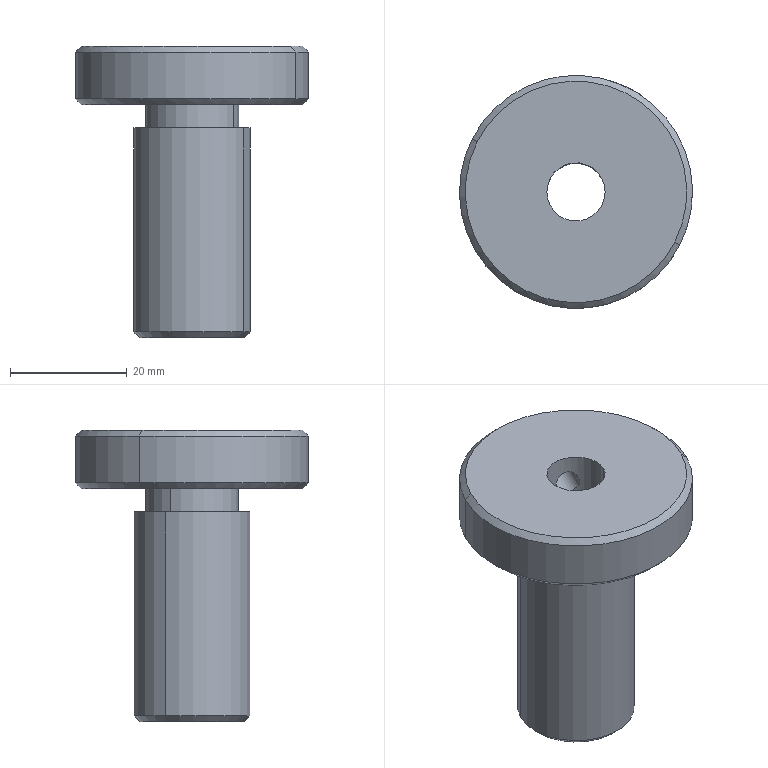Component | SolidWorks | AdjustingScrew-1 | 1 solid | 20 faces | box 40 x 40 x 50 mm | volume 20390 mm3 | cylinder 10 | cone 6 | plane 4 | commonest cylinder face diameters 4.2 x2 10 x2 40 x2 16 x2 20 x2
build123d program:
from build123d import *

# Parameters (mm, degrees)
F_10_0_10_DIAMETER_HOLE1_D = 10
SKETCH4_W                  = 2.1
SKETCH4_H                  = 15.462


with BuildPart() as part:
    # Sketch1 → Revolve1 (revolve)
    with BuildSketch(Plane.XY, mode=Mode.PRIVATE) as revolve1_sk:
        Polygon((-50, 9), (-50, 0), (0, 0), (0, 19), (-1, 20), (-9, 20), (-10, 19), (-10, 8), (-14, 8), (-14, 10), (-49, 10), align=None)
    revolve(revolve1_sk.sketch.rotate(Axis((-50, 0, 0), (1, 0, 0)), 270), axis=Axis((-50, 0, 0), (1, 0, 0)))

    # 10.0 _10_ Diameter Hole1 (through all)
    with Locations(Plane.ZY.offset(50)):
        with Locations((0, 0)):
            Hole(F_10_0_10_DIAMETER_HOLE1_D / 2)

    # Sketch4 → 4.2 _4.2_ Diameter Hole1 (revolve, cut)
    with BuildSketch(Plane(origin=(-5, 4.538, 0), x_dir=(0, 0, -1), z_dir=(1, 0, 0))):
        with Locations((1.05, 7.731)):
            Rectangle(SKETCH4_W, SKETCH4_H)
    revolve(axis=Axis((-5, -1.812, 0), (0, 1, 0)), mode=Mode.SUBTRACT)


solid = part.part

# Placed as in the assembly
solid = solid.moved(Location((376.258, 489.105, 284.94), (-90, -63.116, -90)))
STEP:
#1=COLOUR_RGB('',0.7922,0.8196,0.9333);
#2=FILL_AREA_STYLE_COLOUR('',#1);
#3=FILL_AREA_STYLE('',(#2));
#4=SURFACE_STYLE_FILL_AREA(#3);
#5=SURFACE_SIDE_STYLE('',(#4));
#6=SURFACE_STYLE_USAGE(.BOTH.,#5);
#7=PRESENTATION_STYLE_ASSIGNMENT((#6));
#8=CARTESIAN_POINT('',(15.241,19.917,11.021));
#9=VERTEX_POINT('',#8);
#10=CARTESIAN_POINT('',(15.094,19.992,11.021));
#11=VERTEX_POINT('',#10);
#12=CARTESIAN_POINT('',(15.241,19.917,11.021));
#13=CARTESIAN_POINT('',(15.241,19.917,11.016));
#14=CARTESIAN_POINT('',(15.241,19.917,11.01));
#15=CARTESIAN_POINT('',(15.239,19.919,11.));
#16=CARTESIAN_POINT('',(15.238,19.919,10.995));
#17=CARTESIAN_POINT('',(15.234,19.922,10.985));
#18=CARTESIAN_POINT('',(15.232,19.923,10.98));
#19=CARTESIAN_POINT('',(15.227,19.926,10.971));
#20=CARTESIAN_POINT('',(15.224,19.928,10.967));
#21=CARTESIAN_POINT('',(15.217,19.932,10.959));
#22=CARTESIAN_POINT('',(15.214,19.934,10.956));
#23=CARTESIAN_POINT('',(15.206,19.939,10.95));
#24=CARTESIAN_POINT('',(15.202,19.941,10.947));
#25=CARTESIAN_POINT('',(15.193,19.946,10.943));
#26=CARTESIAN_POINT('',(15.188,19.948,10.941));
#27=CARTESIAN_POINT('',(15.179,19.953,10.939));
#28=CARTESIAN_POINT('',(15.174,19.956,10.939));
#29=CARTESIAN_POINT('',(15.16,19.963,10.939));
#30=CARTESIAN_POINT('',(15.15,19.968,10.941));
#31=CARTESIAN_POINT('',(15.132,19.976,10.949));
#32=CARTESIAN_POINT('',(15.123,19.98,10.955));
#33=CARTESIAN_POINT('',(15.113,19.984,10.967));
#34=CARTESIAN_POINT('',(15.109,19.986,10.971));
#35=CARTESIAN_POINT('',(15.104,19.988,10.98));
#36=CARTESIAN_POINT('',(15.102,19.989,10.985));
#37=CARTESIAN_POINT('',(15.098,19.99,10.995));
#38=CARTESIAN_POINT('',(15.096,19.991,11.));
#39=CARTESIAN_POINT('',(15.094,19.992,11.01));
#40=CARTESIAN_POINT('',(15.094,19.992,11.016));
#41=CARTESIAN_POINT('',(15.094,19.992,11.021));
#42=B_SPLINE_CURVE_WITH_KNOTS('',3,(#12,#13,#14,#15,#16,#17,#18,#19,#20,#21,#22,#23,#24,#25,#26,#27,#28,#29,#30,#31,#32,#33,#34,#35,#36,#37,#38,#39,#40,#41),.UNSPECIFIED.,.F.,.F.,(4,2,2,2,2,2,2,2,2,2,2,2,2,2,4),(0.003286,0.003696,0.004107,0.004518,0.004928,0.005339,0.00575,0.00616,0.006571,0.007392,0.008213,0.008624,0.009035,0.009445,0.009856),.UNSPECIFIED.);
#43=EDGE_CURVE('',#9,#11,#42,.T.);
#44=ORIENTED_EDGE('',*,*,#43,.T.);
#45=CARTESIAN_POINT('',(14.82,19.453,11.021));
#46=VERTEX_POINT('',#45);
#47=CARTESIAN_POINT('',(14.82,19.453,11.021));
#48=DIRECTION('',(-0.4522,-0.8919,-0.));
#49=VECTOR('',#48,39.37);
#50=LINE('',#47,#49);
#51=EDGE_CURVE('',#11,#46,#50,.T.);
#52=ORIENTED_EDGE('',*,*,#51,.T.);
#53=CARTESIAN_POINT('',(14.968,19.378,11.021));
#54=VERTEX_POINT('',#53);
#55=CARTESIAN_POINT('',(14.968,19.378,11.021));
#56=CARTESIAN_POINT('',(14.968,19.378,11.016));
#57=CARTESIAN_POINT('',(14.967,19.379,11.01));
#58=CARTESIAN_POINT('',(14.966,19.38,11.));
#59=CARTESIAN_POINT('',(14.965,19.382,10.994));
#60=CARTESIAN_POINT('',(14.962,19.385,10.984));
#61=CARTESIAN_POINT('',(14.96,19.387,10.98));
#62=CARTESIAN_POINT('',(14.956,19.392,10.971));
#63=CARTESIAN_POINT('',(14.953,19.395,10.967));
#64=CARTESIAN_POINT('',(14.945,19.403,10.955));
#65=CARTESIAN_POINT('',(14.938,19.409,10.949));
#66=CARTESIAN_POINT('',(14.926,19.418,10.943));
#67=CARTESIAN_POINT('',(14.921,19.421,10.941));
#68=CARTESIAN_POINT('',(14.912,19.427,10.939));
#69=CARTESIAN_POINT('',(14.907,19.429,10.939));
#70=CARTESIAN_POINT('',(14.897,19.434,10.939));
#71=CARTESIAN_POINT('',(14.892,19.436,10.939));
#72=CARTESIAN_POINT('',(14.883,19.44,10.941));
#73=CARTESIAN_POINT('',(14.878,19.442,10.943));
#74=CARTESIAN_POINT('',(14.868,19.445,10.947));
#75=CARTESIAN_POINT('',(14.863,19.447,10.95));
#76=CARTESIAN_POINT('',(14.854,19.449,10.956));
#77=CARTESIAN_POINT('',(14.85,19.45,10.959));
#78=CARTESIAN_POINT('',(14.842,19.451,10.967));
#79=CARTESIAN_POINT('',(14.839,19.451,10.971));
#80=CARTESIAN_POINT('',(14.832,19.452,10.98));
#81=CARTESIAN_POINT('',(14.83,19.452,10.984));
#82=CARTESIAN_POINT('',(14.823,19.453,10.999));
#83=CARTESIAN_POINT('',(14.82,19.453,11.01));
#84=CARTESIAN_POINT('',(14.82,19.453,11.021));
#85=B_SPLINE_CURVE_WITH_KNOTS('',3,(#55,#56,#57,#58,#59,#60,#61,#62,#63,#64,#65,#66,#67,#68,#69,#70,#71,#72,#73,#74,#75,#76,#77,#78,#79,#80,#81,#82,#83,#84),.UNSPECIFIED.,.F.,.F.,(4,2,2,2,2,2,2,2,2,2,2,2,2,2,4),(0.,0.0004152,0.0008304,0.001246,0.001661,0.002491,0.002906,0.003322,0.003737,0.004152,0.004567,0.004982,0.005398,0.005813,0.006643),.UNSPECIFIED.);
#86=EDGE_CURVE('',#54,#46,#85,.T.);
#87=ORIENTED_EDGE('',*,*,#86,.F.);
#88=CARTESIAN_POINT('',(14.968,19.378,11.021));
#89=DIRECTION('',(-0.4522,-0.8919,-0.));
#90=VECTOR('',#89,39.37);
#91=LINE('',#88,#90);
#92=EDGE_CURVE('',#9,#54,#91,.T.);
#93=ORIENTED_EDGE('',*,*,#92,.F.);
#94=EDGE_LOOP('',(#44,#52,#87,#93));
#95=FACE_OUTER_BOUND('',#94,.T.);
#96=CARTESIAN_POINT('',(14.894,19.415,11.021));
#97=DIRECTION('',(-0.4522,-0.8919,-0.));
#98=DIRECTION('',(0.8919,-0.4522,0.));
#99=AXIS2_PLACEMENT_3D('',#96,#97,#98);
#100=CYLINDRICAL_SURFACE('',#99,0.08268);
#101=ADVANCED_FACE('',(#95),#100,.F.);
#102=CARTESIAN_POINT('',(14.989,19.167,11.218));
#103=VERTEX_POINT('',#102);
#104=CARTESIAN_POINT('',(14.638,19.345,11.218));
#105=VERTEX_POINT('',#104);
#106=CARTESIAN_POINT('',(14.813,19.256,11.218));
#107=DIRECTION('',(0.,0.,-1.));
#108=DIRECTION('',(-0.8919,0.4522,0.));
#109=AXIS2_PLACEMENT_3D('',#106,#107,#108);
#110=CIRCLE('',#109,0.1969);
#111=EDGE_CURVE('',#103,#105,#110,.T.);
#112=ORIENTED_EDGE('',*,*,#111,.F.);
#113=CARTESIAN_POINT('',(14.989,19.167,9.25));
#114=VERTEX_POINT('',#113);
#115=CARTESIAN_POINT('',(14.989,19.167,9.25));
#116=DIRECTION('',(0.,0.,-1.));
#117=VECTOR('',#116,39.37);
#118=LINE('',#115,#117);
#119=EDGE_CURVE('',#103,#114,#118,.T.);
#120=ORIENTED_EDGE('',*,*,#119,.T.);
#121=CARTESIAN_POINT('',(14.638,19.345,9.25));
#122=VERTEX_POINT('',#121);
#123=CARTESIAN_POINT('',(14.813,19.256,9.25));
#124=DIRECTION('',(0.,0.,-1.));
#125=DIRECTION('',(-0.8919,0.4522,0.));
#126=AXIS2_PLACEMENT_3D('',#123,#124,#125);
#127=CIRCLE('',#126,0.1969);
#128=EDGE_CURVE('',#114,#122,#127,.T.);
#129=ORIENTED_EDGE('',*,*,#128,.T.);
#130=CARTESIAN_POINT('',(14.638,19.345,9.25));
#131=DIRECTION('',(0.,0.,-1.));
#132=VECTOR('',#131,39.37);
#133=LINE('',#130,#132);
#134=EDGE_CURVE('',#105,#122,#133,.T.);
#135=ORIENTED_EDGE('',*,*,#134,.F.);
#136=EDGE_LOOP('',(#112,#120,#129,#135));
#137=FACE_OUTER_BOUND('',#136,.T.);
#138=CARTESIAN_POINT('',(14.813,19.256,9.25));
#139=DIRECTION('',(0.,0.,-1.));
#140=DIRECTION('',(-0.8919,0.4522,0.));
#141=AXIS2_PLACEMENT_3D('',#138,#139,#140);
#142=CYLINDRICAL_SURFACE('',#141,0.1969);
#143=ADVANCED_FACE('',(#137),#142,.F.);
#144=CARTESIAN_POINT('',(15.48,18.918,11.218));
#145=VERTEX_POINT('',#144);
#146=CARTESIAN_POINT('',(14.146,19.594,11.218));
#147=VERTEX_POINT('',#146);
#148=CARTESIAN_POINT('',(14.813,19.256,11.218));
#149=DIRECTION('',(-0.,-0.,1.));
#150=DIRECTION('',(0.8919,-0.4522,0.));
#151=AXIS2_PLACEMENT_3D('',#148,#149,#150);
#152=CIRCLE('',#151,0.748);
#153=EDGE_CURVE('',#145,#147,#152,.T.);
#154=ORIENTED_EDGE('',*,*,#153,.F.);
#155=CARTESIAN_POINT('',(15.516,18.9,11.179));
#156=VERTEX_POINT('',#155);
#157=CARTESIAN_POINT('',(15.48,18.918,11.218));
#158=DIRECTION('',(0.6307,-0.3198,-0.7071));
#159=VECTOR('',#158,39.37);
#160=LINE('',#157,#159);
#161=EDGE_CURVE('',#145,#156,#160,.T.);
#162=ORIENTED_EDGE('',*,*,#161,.T.);
#163=CARTESIAN_POINT('',(14.111,19.612,11.179));
#164=VERTEX_POINT('',#163);
#165=CARTESIAN_POINT('',(14.813,19.256,11.179));
#166=DIRECTION('',(-0.,-0.,1.));
#167=DIRECTION('',(0.8919,-0.4522,0.));
#168=AXIS2_PLACEMENT_3D('',#165,#166,#167);
#169=CIRCLE('',#168,0.7874);
#170=EDGE_CURVE('',#156,#164,#169,.T.);
#171=ORIENTED_EDGE('',*,*,#170,.T.);
#172=CARTESIAN_POINT('',(14.146,19.594,11.218));
#173=DIRECTION('',(-0.6307,0.3198,-0.7071));
#174=VECTOR('',#173,39.37);
#175=LINE('',#172,#174);
#176=EDGE_CURVE('',#147,#164,#175,.T.);
#177=ORIENTED_EDGE('',*,*,#176,.F.);
#178=EDGE_LOOP('',(#154,#162,#171,#177));
#179=FACE_OUTER_BOUND('',#178,.T.);
#180=CARTESIAN_POINT('',(14.813,19.256,11.218));
#181=DIRECTION('',(0.,0.,-1.));
#182=DIRECTION('',(-0.8919,0.4522,0.));
#183=AXIS2_PLACEMENT_3D('',#180,#181,#182);
#184=CONICAL_SURFACE('',#183,0.748,0.7854);
#185=ADVANCED_FACE('',(#179),#184,.T.);
#186=ORIENTED_EDGE('',*,*,#43,.F.);
#187=CARTESIAN_POINT('',(15.094,19.992,11.021));
#188=CARTESIAN_POINT('',(15.094,19.992,11.027));
#189=CARTESIAN_POINT('',(15.094,19.992,11.032));
#190=CARTESIAN_POINT('',(15.096,19.991,11.043));
#191=CARTESIAN_POINT('',(15.098,19.99,11.048));
#192=CARTESIAN_POINT('',(15.102,19.989,11.058));
#193=CARTESIAN_POINT('',(15.104,19.988,11.063));
#194=CARTESIAN_POINT('',(15.109,19.986,11.072));
#195=CARTESIAN_POINT('',(15.113,19.984,11.076));
#196=CARTESIAN_POINT('',(15.123,19.98,11.087));
#197=CARTESIAN_POINT('',(15.132,19.976,11.094));
#198=CARTESIAN_POINT('',(15.15,19.968,11.102));
#199=CARTESIAN_POINT('',(15.16,19.963,11.104));
#200=CARTESIAN_POINT('',(15.174,19.956,11.104));
#201=CARTESIAN_POINT('',(15.179,19.953,11.103));
#202=CARTESIAN_POINT('',(15.188,19.948,11.101));
#203=CARTESIAN_POINT('',(15.193,19.946,11.1));
#204=CARTESIAN_POINT('',(15.202,19.941,11.096));
#205=CARTESIAN_POINT('',(15.206,19.939,11.093));
#206=CARTESIAN_POINT('',(15.214,19.934,11.087));
#207=CARTESIAN_POINT('',(15.217,19.932,11.083));
#208=CARTESIAN_POINT('',(15.227,19.926,11.072));
#209=CARTESIAN_POINT('',(15.232,19.923,11.063));
#210=CARTESIAN_POINT('',(15.239,19.918,11.043));
#211=CARTESIAN_POINT('',(15.241,19.917,11.032));
#212=CARTESIAN_POINT('',(15.241,19.917,11.021));
#213=B_SPLINE_CURVE_WITH_KNOTS('',3,(#187,#188,#189,#190,#191,#192,#193,#194,#195,#196,#197,#198,#199,#200,#201,#202,#203,#204,#205,#206,#207,#208,#209,#210,#211,#212),.UNSPECIFIED.,.F.,.F.,(4,2,2,2,2,2,2,2,2,2,2,2,4),(0.009856,0.01027,0.01068,0.01109,0.0115,0.01232,0.01314,0.01355,0.01396,0.01437,0.01478,0.0156,0.01642),.UNSPECIFIED.);
#214=EDGE_CURVE('',#11,#9,#213,.T.);
#215=ORIENTED_EDGE('',*,*,#214,.F.);
#216=EDGE_LOOP('',(#186,#215));
#217=FACE_BOUND('',#216,.T.);
#218=CARTESIAN_POINT('',(15.516,18.9,10.864));
#219=VERTEX_POINT('',#218);
#220=CARTESIAN_POINT('',(14.111,19.612,10.864));
#221=VERTEX_POINT('',#220);
#222=CARTESIAN_POINT('',(14.813,19.256,10.864));
#223=DIRECTION('',(-0.,-0.,1.));
#224=DIRECTION('',(0.8919,-0.4522,0.));
#225=AXIS2_PLACEMENT_3D('',#222,#223,#224);
#226=CIRCLE('',#225,0.7874);
#227=EDGE_CURVE('',#219,#221,#226,.T.);
#228=ORIENTED_EDGE('',*,*,#227,.T.);
#229=CARTESIAN_POINT('',(14.111,19.612,9.25));
#230=DIRECTION('',(-0.,-0.,1.));
#231=VECTOR('',#230,39.37);
#232=LINE('',#229,#231);
#233=EDGE_CURVE('',#221,#164,#232,.T.);
#234=ORIENTED_EDGE('',*,*,#233,.T.);
#235=ORIENTED_EDGE('',*,*,#170,.F.);
#236=CARTESIAN_POINT('',(15.516,18.9,9.25));
#237=DIRECTION('',(-0.,-0.,1.));
#238=VECTOR('',#237,39.37);
#239=LINE('',#236,#238);
#240=EDGE_CURVE('',#219,#156,#239,.T.);
#241=ORIENTED_EDGE('',*,*,#240,.F.);
#242=EDGE_LOOP('',(#228,#234,#235,#241));
#243=FACE_OUTER_BOUND('',#242,.T.);
#244=CARTESIAN_POINT('',(14.813,19.256,9.25));
#245=DIRECTION('',(-0.,-0.,1.));
#246=DIRECTION('',(0.8919,-0.4522,0.));
#247=AXIS2_PLACEMENT_3D('',#244,#245,#246);
#248=CYLINDRICAL_SURFACE('',#247,0.7874);
#249=ADVANCED_FACE('',(#217,#243),#248,.T.);
#250=CARTESIAN_POINT('',(15.48,18.918,10.824));
#251=VERTEX_POINT('',#250);
#252=CARTESIAN_POINT('',(14.146,19.594,10.824));
#253=VERTEX_POINT('',#252);
#254=CARTESIAN_POINT('',(14.813,19.256,10.824));
#255=DIRECTION('',(-0.,-0.,1.));
#256=DIRECTION('',(0.8919,-0.4522,0.));
#257=AXIS2_PLACEMENT_3D('',#254,#255,#256);
#258=CIRCLE('',#257,0.748);
#259=EDGE_CURVE('',#251,#253,#258,.T.);
#260=ORIENTED_EDGE('',*,*,#259,.T.);
#261=CARTESIAN_POINT('',(14.111,19.612,10.864));
#262=DIRECTION('',(-0.6307,0.3198,0.7071));
#263=VECTOR('',#262,39.37);
#264=LINE('',#261,#263);
#265=EDGE_CURVE('',#253,#221,#264,.T.);
#266=ORIENTED_EDGE('',*,*,#265,.T.);
#267=ORIENTED_EDGE('',*,*,#227,.F.);
#268=CARTESIAN_POINT('',(15.516,18.9,10.864));
#269=DIRECTION('',(0.6307,-0.3198,0.7071));
#270=VECTOR('',#269,39.37);
#271=LINE('',#268,#270);
#272=EDGE_CURVE('',#251,#219,#271,.T.);
#273=ORIENTED_EDGE('',*,*,#272,.F.);
#274=EDGE_LOOP('',(#260,#266,#267,#273));
#275=FACE_OUTER_BOUND('',#274,.T.);
#276=CARTESIAN_POINT('',(14.813,19.256,10.864));
#277=DIRECTION('',(-0.,-0.,1.));
#278=DIRECTION('',(0.8919,-0.4522,0.));
#279=AXIS2_PLACEMENT_3D('',#276,#277,#278);
#280=CONICAL_SURFACE('',#279,0.7874,0.7854);
#281=ADVANCED_FACE('',(#275),#280,.T.);
#282=CARTESIAN_POINT('',(15.094,19.114,10.667));
#283=VERTEX_POINT('',#282);
#284=CARTESIAN_POINT('',(14.532,19.399,10.667));
#285=VERTEX_POINT('',#284);
#286=CARTESIAN_POINT('',(14.813,19.256,10.667));
#287=DIRECTION('',(-0.,-0.,1.));
#288=DIRECTION('',(0.8919,-0.4522,0.));
#289=AXIS2_PLACEMENT_3D('',#286,#287,#288);
#290=CIRCLE('',#289,0.315);
#291=EDGE_CURVE('',#283,#285,#290,.T.);
#292=ORIENTED_EDGE('',*,*,#291,.T.);
#293=CARTESIAN_POINT('',(14.532,19.399,10.824));
#294=VERTEX_POINT('',#293);
#295=CARTESIAN_POINT('',(14.532,19.399,9.25));
#296=DIRECTION('',(-0.,-0.,1.));
#297=VECTOR('',#296,39.37);
#298=LINE('',#295,#297);
#299=EDGE_CURVE('',#285,#294,#298,.T.);
#300=ORIENTED_EDGE('',*,*,#299,.T.);
#301=CARTESIAN_POINT('',(15.094,19.114,10.824));
#302=VERTEX_POINT('',#301);
#303=CARTESIAN_POINT('',(14.813,19.256,10.824));
#304=DIRECTION('',(-0.,-0.,1.));
#305=DIRECTION('',(0.8919,-0.4522,0.));
#306=AXIS2_PLACEMENT_3D('',#303,#304,#305);
#307=CIRCLE('',#306,0.315);
#308=EDGE_CURVE('',#302,#294,#307,.T.);
#309=ORIENTED_EDGE('',*,*,#308,.F.);
#310=CARTESIAN_POINT('',(15.094,19.114,9.25));
#311=DIRECTION('',(-0.,-0.,1.));
#312=VECTOR('',#311,39.37);
#313=LINE('',#310,#312);
#314=EDGE_CURVE('',#283,#302,#313,.T.);
#315=ORIENTED_EDGE('',*,*,#314,.F.);
#316=EDGE_LOOP('',(#292,#300,#309,#315));
#317=FACE_OUTER_BOUND('',#316,.T.);
#318=CARTESIAN_POINT('',(14.813,19.256,9.25));
#319=DIRECTION('',(-0.,-0.,1.));
#320=DIRECTION('',(0.8919,-0.4522,0.));
#321=AXIS2_PLACEMENT_3D('',#318,#319,#320);
#322=CYLINDRICAL_SURFACE('',#321,0.315);
#323=ADVANCED_FACE('',(#317),#322,.T.);
#324=CARTESIAN_POINT('',(15.164,19.078,9.289));
#325=VERTEX_POINT('',#324);
#326=CARTESIAN_POINT('',(14.462,19.434,9.289));
#327=VERTEX_POINT('',#326);
#328=CARTESIAN_POINT('',(14.813,19.256,9.289));
#329=DIRECTION('',(-0.,-0.,1.));
#330=DIRECTION('',(0.8919,-0.4522,0.));
#331=AXIS2_PLACEMENT_3D('',#328,#329,#330);
#332=CIRCLE('',#331,0.3937);
#333=EDGE_CURVE('',#325,#327,#332,.T.);
#334=ORIENTED_EDGE('',*,*,#333,.T.);
#335=CARTESIAN_POINT('',(14.462,19.434,10.667));
#336=VERTEX_POINT('',#335);
#337=CARTESIAN_POINT('',(14.462,19.434,9.25));
#338=DIRECTION('',(-0.,-0.,1.));
#339=VECTOR('',#338,39.37);
#340=LINE('',#337,#339);
#341=EDGE_CURVE('',#327,#336,#340,.T.);
#342=ORIENTED_EDGE('',*,*,#341,.T.);
#343=CARTESIAN_POINT('',(15.164,19.078,10.667));
#344=VERTEX_POINT('',#343);
#345=CARTESIAN_POINT('',(14.813,19.256,10.667));
#346=DIRECTION('',(-0.,-0.,1.));
#347=DIRECTION('',(0.8919,-0.4522,0.));
#348=AXIS2_PLACEMENT_3D('',#345,#346,#347);
#349=CIRCLE('',#348,0.3937);
#350=EDGE_CURVE('',#344,#336,#349,.T.);
#351=ORIENTED_EDGE('',*,*,#350,.F.);
#352=CARTESIAN_POINT('',(15.164,19.078,9.25));
#353=DIRECTION('',(-0.,-0.,1.));
#354=VECTOR('',#353,39.37);
#355=LINE('',#352,#354);
#356=EDGE_CURVE('',#325,#344,#355,.T.);
#357=ORIENTED_EDGE('',*,*,#356,.F.);
#358=EDGE_LOOP('',(#334,#342,#351,#357));
#359=FACE_OUTER_BOUND('',#358,.T.);
#360=CARTESIAN_POINT('',(14.813,19.256,9.25));
#361=DIRECTION('',(-0.,-0.,1.));
#362=DIRECTION('',(0.8919,-0.4522,0.));
#363=AXIS2_PLACEMENT_3D('',#360,#361,#362);
#364=CYLINDRICAL_SURFACE('',#363,0.3937);
#365=ADVANCED_FACE('',(#359),#364,.T.);
#366=CARTESIAN_POINT('',(15.129,19.096,9.25));
#367=VERTEX_POINT('',#366);
#368=CARTESIAN_POINT('',(14.497,19.416,9.25));
#369=VERTEX_POINT('',#368);
#370=CARTESIAN_POINT('',(14.813,19.256,9.25));
#371=DIRECTION('',(-0.,-0.,1.));
#372=DIRECTION('',(0.8919,-0.4522,0.));
#373=AXIS2_PLACEMENT_3D('',#370,#371,#372);
#374=CIRCLE('',#373,0.3543);
#375=EDGE_CURVE('',#367,#369,#374,.T.);
#376=ORIENTED_EDGE('',*,*,#375,.T.);
#377=CARTESIAN_POINT('',(14.462,19.434,9.289));
#378=DIRECTION('',(-0.6307,0.3198,0.7071));
#379=VECTOR('',#378,39.37);
#380=LINE('',#377,#379);
#381=EDGE_CURVE('',#369,#327,#380,.T.);
#382=ORIENTED_EDGE('',*,*,#381,.T.);
#383=ORIENTED_EDGE('',*,*,#333,.F.);
#384=CARTESIAN_POINT('',(15.164,19.078,9.289));
#385=DIRECTION('',(0.6307,-0.3198,0.7071));
#386=VECTOR('',#385,39.37);
#387=LINE('',#384,#386);
#388=EDGE_CURVE('',#367,#325,#387,.T.);
#389=ORIENTED_EDGE('',*,*,#388,.F.);
#390=EDGE_LOOP('',(#376,#382,#383,#389));
#391=FACE_OUTER_BOUND('',#390,.T.);
#392=CARTESIAN_POINT('',(14.813,19.256,9.289));
#393=DIRECTION('',(-0.,-0.,1.));
#394=DIRECTION('',(0.8919,-0.4522,0.));
#395=AXIS2_PLACEMENT_3D('',#392,#393,#394);
#396=CONICAL_SURFACE('',#395,0.3937,0.7854);
#397=ADVANCED_FACE('',(#391),#396,.T.);
#398=CARTESIAN_POINT('',(14.813,19.256,11.218));
#399=DIRECTION('',(-0.,-0.,1.));
#400=DIRECTION('',(0.8919,-0.4522,0.));
#401=AXIS2_PLACEMENT_3D('',#398,#399,#400);
#402=CIRCLE('',#401,0.748);
#403=EDGE_CURVE('',#147,#145,#402,.T.);
#404=ORIENTED_EDGE('',*,*,#403,.T.);
#405=ORIENTED_EDGE('',*,*,#153,.T.);
#406=EDGE_LOOP('',(#404,#405));
#407=FACE_OUTER_BOUND('',#406,.T.);
#408=CARTESIAN_POINT('',(14.813,19.256,11.218));
#409=DIRECTION('',(0.,0.,-1.));
#410=DIRECTION('',(-0.8919,0.4522,0.));
#411=AXIS2_PLACEMENT_3D('',#408,#409,#410);
#412=CIRCLE('',#411,0.1969);
#413=EDGE_CURVE('',#105,#103,#412,.T.);
#414=ORIENTED_EDGE('',*,*,#413,.T.);
#415=ORIENTED_EDGE('',*,*,#111,.T.);
#416=EDGE_LOOP('',(#414,#415));
#417=FACE_BOUND('',#416,.T.);
#418=CARTESIAN_POINT('',(14.813,19.256,11.218));
#419=DIRECTION('',(-0.,-0.,1.));
#420=DIRECTION('',(0.8919,-0.4522,0.));
#421=AXIS2_PLACEMENT_3D('',#418,#419,#420);
#422=PLANE('',#421);
#423=ADVANCED_FACE('',(#407,#417),#422,.T.);
#424=ORIENTED_EDGE('',*,*,#381,.F.);
#425=CARTESIAN_POINT('',(14.813,19.256,9.25));
#426=DIRECTION('',(-0.,-0.,1.));
#427=DIRECTION('',(0.8919,-0.4522,0.));
#428=AXIS2_PLACEMENT_3D('',#425,#426,#427);
#429=CIRCLE('',#428,0.3543);
#430=EDGE_CURVE('',#369,#367,#429,.T.);
#431=ORIENTED_EDGE('',*,*,#430,.T.);
#432=ORIENTED_EDGE('',*,*,#388,.T.);
#433=CARTESIAN_POINT('',(14.813,19.256,9.289));
#434=DIRECTION('',(-0.,-0.,1.));
#435=DIRECTION('',(0.8919,-0.4522,0.));
#436=AXIS2_PLACEMENT_3D('',#433,#434,#435);
#437=CIRCLE('',#436,0.3937);
#438=EDGE_CURVE('',#327,#325,#437,.T.);
#439=ORIENTED_EDGE('',*,*,#438,.F.);
#440=EDGE_LOOP('',(#424,#431,#432,#439));
#441=FACE_OUTER_BOUND('',#440,.T.);
#442=CARTESIAN_POINT('',(14.813,19.256,9.289));
#443=DIRECTION('',(-0.,-0.,1.));
#444=DIRECTION('',(0.8919,-0.4522,0.));
#445=AXIS2_PLACEMENT_3D('',#442,#443,#444);
#446=CONICAL_SURFACE('',#445,0.3937,0.7854);
#447=ADVANCED_FACE('',(#441),#446,.T.);
#448=ORIENTED_EDGE('',*,*,#341,.F.);
#449=ORIENTED_EDGE('',*,*,#438,.T.);
#450=ORIENTED_EDGE('',*,*,#356,.T.);
#451=CARTESIAN_POINT('',(14.813,19.256,10.667));
#452=DIRECTION('',(-0.,-0.,1.));
#453=DIRECTION('',(0.8919,-0.4522,0.));
#454=AXIS2_PLACEMENT_3D('',#451,#452,#453);
#455=CIRCLE('',#454,0.3937);
#456=EDGE_CURVE('',#336,#344,#455,.T.);
#457=ORIENTED_EDGE('',*,*,#456,.F.);
#458=EDGE_LOOP('',(#448,#449,#450,#457));
#459=FACE_OUTER_BOUND('',#458,.T.);
#460=CARTESIAN_POINT('',(14.813,19.256,9.25));
#461=DIRECTION('',(-0.,-0.,1.));
#462=DIRECTION('',(0.8919,-0.4522,0.));
#463=AXIS2_PLACEMENT_3D('',#460,#461,#462);
#464=CYLINDRICAL_SURFACE('',#463,0.3937);
#465=ADVANCED_FACE('',(#459),#464,.T.);
#466=ORIENTED_EDGE('',*,*,#350,.T.);
#467=ORIENTED_EDGE('',*,*,#456,.T.);
#468=EDGE_LOOP('',(#466,#467));
#469=FACE_OUTER_BOUND('',#468,.T.);
#470=ORIENTED_EDGE('',*,*,#291,.F.);
#471=CARTESIAN_POINT('',(14.813,19.256,10.667));
#472=DIRECTION('',(-0.,-0.,1.));
#473=DIRECTION('',(0.8919,-0.4522,0.));
#474=AXIS2_PLACEMENT_3D('',#471,#472,#473);
#475=CIRCLE('',#474,0.315);
#476=EDGE_CURVE('',#285,#283,#475,.T.);
#477=ORIENTED_EDGE('',*,*,#476,.F.);
#478=EDGE_LOOP('',(#470,#477));
#479=FACE_BOUND('',#478,.T.);
#480=CARTESIAN_POINT('',(14.956,19.537,10.667));
#481=DIRECTION('',(-0.,-0.,1.));
#482=DIRECTION('',(0.8919,-0.4522,0.));
#483=AXIS2_PLACEMENT_3D('',#480,#481,#482);
#484=PLANE('',#483);
#485=ADVANCED_FACE('',(#469,#479),#484,.T.);
#486=ORIENTED_EDGE('',*,*,#299,.F.);
#487=ORIENTED_EDGE('',*,*,#476,.T.);
#488=ORIENTED_EDGE('',*,*,#314,.T.);
#489=CARTESIAN_POINT('',(14.813,19.256,10.824));
#490=DIRECTION('',(-0.,-0.,1.));
#491=DIRECTION('',(0.8919,-0.4522,0.));
#492=AXIS2_PLACEMENT_3D('',#489,#490,#491);
#493=CIRCLE('',#492,0.315);
#494=EDGE_CURVE('',#294,#302,#493,.T.);
#495=ORIENTED_EDGE('',*,*,#494,.F.);
#496=EDGE_LOOP('',(#486,#487,#488,#495));
#497=FACE_OUTER_BOUND('',#496,.T.);
#498=CARTESIAN_POINT('',(14.813,19.256,9.25));
#499=DIRECTION('',(-0.,-0.,1.));
#500=DIRECTION('',(0.8919,-0.4522,0.));
#501=AXIS2_PLACEMENT_3D('',#498,#499,#500);
#502=CYLINDRICAL_SURFACE('',#501,0.315);
#503=ADVANCED_FACE('',(#497),#502,.T.);
#504=ORIENTED_EDGE('',*,*,#308,.T.);
#505=ORIENTED_EDGE('',*,*,#494,.T.);
#506=EDGE_LOOP('',(#504,#505));
#507=FACE_BOUND('',#506,.T.);
#508=ORIENTED_EDGE('',*,*,#259,.F.);
#509=CARTESIAN_POINT('',(14.813,19.256,10.824));
#510=DIRECTION('',(-0.,-0.,1.));
#511=DIRECTION('',(0.8919,-0.4522,0.));
#512=AXIS2_PLACEMENT_3D('',#509,#510,#511);
#513=CIRCLE('',#512,0.748);
#514=EDGE_CURVE('',#253,#251,#513,.T.);
#515=ORIENTED_EDGE('',*,*,#514,.F.);
#516=EDGE_LOOP('',(#508,#515));
#517=FACE_OUTER_BOUND('',#516,.T.);
#518=CARTESIAN_POINT('',(15.152,19.923,10.824));
#519=DIRECTION('',(0.,0.,-1.));
#520=DIRECTION('',(-0.8919,0.4522,0.));
#521=AXIS2_PLACEMENT_3D('',#518,#519,#520);
#522=PLANE('',#521);
#523=ADVANCED_FACE('',(#507,#517),#522,.T.);
#524=ORIENTED_EDGE('',*,*,#265,.F.);
#525=ORIENTED_EDGE('',*,*,#514,.T.);
#526=ORIENTED_EDGE('',*,*,#272,.T.);
#527=CARTESIAN_POINT('',(14.813,19.256,10.864));
#528=DIRECTION('',(-0.,-0.,1.));
#529=DIRECTION('',(0.8919,-0.4522,0.));
#530=AXIS2_PLACEMENT_3D('',#527,#528,#529);
#531=CIRCLE('',#530,0.7874);
#532=EDGE_CURVE('',#221,#219,#531,.T.);
#533=ORIENTED_EDGE('',*,*,#532,.F.);
#534=EDGE_LOOP('',(#524,#525,#526,#533));
#535=FACE_OUTER_BOUND('',#534,.T.);
#536=CARTESIAN_POINT('',(14.813,19.256,10.864));
#537=DIRECTION('',(-0.,-0.,1.));
#538=DIRECTION('',(0.8919,-0.4522,0.));
#539=AXIS2_PLACEMENT_3D('',#536,#537,#538);
#540=CONICAL_SURFACE('',#539,0.7874,0.7854);
#541=ADVANCED_FACE('',(#535),#540,.T.);
#542=ORIENTED_EDGE('',*,*,#233,.F.);
#543=ORIENTED_EDGE('',*,*,#532,.T.);
#544=ORIENTED_EDGE('',*,*,#240,.T.);
#545=CARTESIAN_POINT('',(14.813,19.256,11.179));
#546=DIRECTION('',(-0.,-0.,1.));
#547=DIRECTION('',(0.8919,-0.4522,0.));
#548=AXIS2_PLACEMENT_3D('',#545,#546,#547);
#549=CIRCLE('',#548,0.7874);
#550=EDGE_CURVE('',#164,#156,#549,.T.);
#551=ORIENTED_EDGE('',*,*,#550,.F.);
#552=EDGE_LOOP('',(#542,#543,#544,#551));
#553=FACE_OUTER_BOUND('',#552,.T.);
#554=CARTESIAN_POINT('',(14.813,19.256,9.25));
#555=DIRECTION('',(-0.,-0.,1.));
#556=DIRECTION('',(0.8919,-0.4522,0.));
#557=AXIS2_PLACEMENT_3D('',#554,#555,#556);
#558=CYLINDRICAL_SURFACE('',#557,0.7874);
#559=ADVANCED_FACE('',(#553),#558,.T.);
#560=ORIENTED_EDGE('',*,*,#161,.F.);
#561=ORIENTED_EDGE('',*,*,#403,.F.);
#562=ORIENTED_EDGE('',*,*,#176,.T.);
#563=ORIENTED_EDGE('',*,*,#550,.T.);
#564=EDGE_LOOP('',(#560,#561,#562,#563));
#565=FACE_OUTER_BOUND('',#564,.T.);
#566=CARTESIAN_POINT('',(14.813,19.256,11.218));
#567=DIRECTION('',(0.,0.,-1.));
#568=DIRECTION('',(-0.8919,0.4522,0.));
#569=AXIS2_PLACEMENT_3D('',#566,#567,#568);
#570=CONICAL_SURFACE('',#569,0.748,0.7854);
#571=ADVANCED_FACE('',(#565),#570,.T.);
#572=CARTESIAN_POINT('',(14.813,19.256,9.25));
#573=DIRECTION('',(0.,0.,-1.));
#574=DIRECTION('',(-0.8919,0.4522,0.));
#575=AXIS2_PLACEMENT_3D('',#572,#573,#574);
#576=CIRCLE('',#575,0.1969);
#577=EDGE_CURVE('',#122,#114,#576,.T.);
#578=ORIENTED_EDGE('',*,*,#577,.F.);
#579=ORIENTED_EDGE('',*,*,#128,.F.);
#580=EDGE_LOOP('',(#578,#579));
#581=FACE_BOUND('',#580,.T.);
#582=ORIENTED_EDGE('',*,*,#375,.F.);
#583=ORIENTED_EDGE('',*,*,#430,.F.);
#584=EDGE_LOOP('',(#582,#583));
#585=FACE_OUTER_BOUND('',#584,.T.);
#586=CARTESIAN_POINT('',(14.974,19.572,9.25));
#587=DIRECTION('',(0.,0.,-1.));
#588=DIRECTION('',(-0.8919,0.4522,0.));
#589=AXIS2_PLACEMENT_3D('',#586,#587,#588);
#590=PLANE('',#589);
#591=ADVANCED_FACE('',(#581,#585),#590,.T.);
#592=ORIENTED_EDGE('',*,*,#119,.F.);
#593=ORIENTED_EDGE('',*,*,#413,.F.);
#594=ORIENTED_EDGE('',*,*,#134,.T.);
#595=ORIENTED_EDGE('',*,*,#577,.T.);
#596=EDGE_LOOP('',(#592,#593,#594,#595));
#597=FACE_OUTER_BOUND('',#596,.T.);
#598=ORIENTED_EDGE('',*,*,#86,.T.);
#599=CARTESIAN_POINT('',(14.82,19.453,11.021));
#600=CARTESIAN_POINT('',(14.82,19.453,11.027));
#601=CARTESIAN_POINT('',(14.821,19.453,11.032));
#602=CARTESIAN_POINT('',(14.823,19.453,11.043));
#603=CARTESIAN_POINT('',(14.825,19.453,11.048));
#604=CARTESIAN_POINT('',(14.832,19.452,11.063));
#605=CARTESIAN_POINT('',(14.838,19.452,11.072));
#606=CARTESIAN_POINT('',(14.85,19.45,11.084));
#607=CARTESIAN_POINT('',(14.854,19.449,11.087));
#608=CARTESIAN_POINT('',(14.863,19.447,11.093));
#609=CARTESIAN_POINT('',(14.868,19.445,11.095));
#610=CARTESIAN_POINT('',(14.878,19.442,11.1));
#611=CARTESIAN_POINT('',(14.882,19.44,11.101));
#612=CARTESIAN_POINT('',(14.892,19.436,11.103));
#613=CARTESIAN_POINT('',(14.897,19.434,11.104));
#614=CARTESIAN_POINT('',(14.912,19.427,11.104));
#615=CARTESIAN_POINT('',(14.921,19.421,11.102));
#616=CARTESIAN_POINT('',(14.934,19.412,11.095));
#617=CARTESIAN_POINT('',(14.937,19.409,11.093));
#618=CARTESIAN_POINT('',(14.944,19.403,11.087));
#619=CARTESIAN_POINT('',(14.948,19.4,11.084));
#620=CARTESIAN_POINT('',(14.953,19.395,11.076));
#621=CARTESIAN_POINT('',(14.956,19.392,11.072));
#622=CARTESIAN_POINT('',(14.96,19.387,11.063));
#623=CARTESIAN_POINT('',(14.962,19.385,11.058));
#624=CARTESIAN_POINT('',(14.965,19.382,11.048));
#625=CARTESIAN_POINT('',(14.966,19.38,11.043));
#626=CARTESIAN_POINT('',(14.967,19.379,11.032));
#627=CARTESIAN_POINT('',(14.968,19.378,11.027));
#628=CARTESIAN_POINT('',(14.968,19.378,11.021));
#629=B_SPLINE_CURVE_WITH_KNOTS('',3,(#599,#600,#601,#602,#603,#604,#605,#606,#607,#608,#609,#610,#611,#612,#613,#614,#615,#616,#617,#618,#619,#620,#621,#622,#623,#624,#625,#626,#627,#628),.UNSPECIFIED.,.F.,.F.,(4,2,2,2,2,2,2,2,2,2,2,2,2,2,4),(0.006643,0.007058,0.007473,0.008303,0.008717,0.009132,0.009547,0.009962,0.01079,0.01121,0.01162,0.01204,0.01245,0.01287,0.01328),.UNSPECIFIED.);
#630=EDGE_CURVE('',#46,#54,#629,.T.);
#631=ORIENTED_EDGE('',*,*,#630,.T.);
#632=EDGE_LOOP('',(#598,#631));
#633=FACE_BOUND('',#632,.T.);
#634=CARTESIAN_POINT('',(14.813,19.256,9.25));
#635=DIRECTION('',(0.,0.,-1.));
#636=DIRECTION('',(-0.8919,0.4522,0.));
#637=AXIS2_PLACEMENT_3D('',#634,#635,#636);
#638=CYLINDRICAL_SURFACE('',#637,0.1969);
#639=ADVANCED_FACE('',(#597,#633),#638,.F.);
#640=ORIENTED_EDGE('',*,*,#51,.F.);
#641=ORIENTED_EDGE('',*,*,#214,.T.);
#642=ORIENTED_EDGE('',*,*,#92,.T.);
#643=ORIENTED_EDGE('',*,*,#630,.F.);
#644=EDGE_LOOP('',(#640,#641,#642,#643));
#645=FACE_OUTER_BOUND('',#644,.T.);
#646=CARTESIAN_POINT('',(14.894,19.415,11.021));
#647=DIRECTION('',(-0.4522,-0.8919,-0.));
#648=DIRECTION('',(0.8919,-0.4522,0.));
#649=AXIS2_PLACEMENT_3D('',#646,#647,#648);
#650=CYLINDRICAL_SURFACE('',#649,0.08268);
#651=ADVANCED_FACE('',(#645),#650,.F.);
#652=CLOSED_SHELL('',(#101,#143,#185,#249,#281,#323,#365,#397,#423,#447,#465,#485,#503,#523,#541,#559,#571,#591,#639,#651));
#653=MANIFOLD_SOLID_BREP('',#652);
#654=STYLED_ITEM('',(#7),#653);
#655=(LENGTH_UNIT()NAMED_UNIT(*)SI_UNIT($,.METRE.));
#656=LENGTH_MEASURE_WITH_UNIT(LENGTH_MEASURE(0.0254),#655);
#657=DIMENSIONAL_EXPONENTS(1.,0.,0.,0.,0.,0.,0.);
#658=(CONVERSION_BASED_UNIT('',#656)LENGTH_UNIT()NAMED_UNIT(#657));
#659=UNCERTAINTY_MEASURE_WITH_UNIT(LENGTH_MEASURE(0.00001),#658,'','');
#660=(NAMED_UNIT(*)PLANE_ANGLE_UNIT()SI_UNIT($,.RADIAN.));
#661=(NAMED_UNIT(*)SI_UNIT($,.STERADIAN.)SOLID_ANGLE_UNIT());
#662=(GEOMETRIC_REPRESENTATION_CONTEXT(3)GLOBAL_UNCERTAINTY_ASSIGNED_CONTEXT((#659))GLOBAL_UNIT_ASSIGNED_CONTEXT((#658,#660,#661))REPRESENTATION_CONTEXT('',''));
#663=MECHANICAL_DESIGN_GEOMETRIC_PRESENTATION_REPRESENTATION('',(#654),#662);
#664=PRESENTATION_LAYER_ASSIGNMENT('','',(#654));
#665=CARTESIAN_POINT('',(0.,0.,0.));
#666=DIRECTION('',(0.,0.,1.));
#667=DIRECTION('',(1.,0.,0.));
#668=AXIS2_PLACEMENT_3D('',#665,#666,#667);
#669=(LENGTH_UNIT()NAMED_UNIT(*)SI_UNIT($,.METRE.));
#670=LENGTH_MEASURE_WITH_UNIT(LENGTH_MEASURE(0.0254),#669);
#671=DIMENSIONAL_EXPONENTS(1.,0.,0.,0.,0.,0.,0.);
#672=(CONVERSION_BASED_UNIT('',#670)LENGTH_UNIT()NAMED_UNIT(#671));
#673=UNCERTAINTY_MEASURE_WITH_UNIT(LENGTH_MEASURE(0.00001),#672,'','');
#674=(NAMED_UNIT(*)PLANE_ANGLE_UNIT()SI_UNIT($,.RADIAN.));
#675=(NAMED_UNIT(*)SI_UNIT($,.STERADIAN.)SOLID_ANGLE_UNIT());
#676=(GEOMETRIC_REPRESENTATION_CONTEXT(3)GLOBAL_UNCERTAINTY_ASSIGNED_CONTEXT((#673))GLOBAL_UNIT_ASSIGNED_CONTEXT((#672,#674,#675))REPRESENTATION_CONTEXT('',''));
#677=ADVANCED_BREP_SHAPE_REPRESENTATION('',(#653,#668),#676);